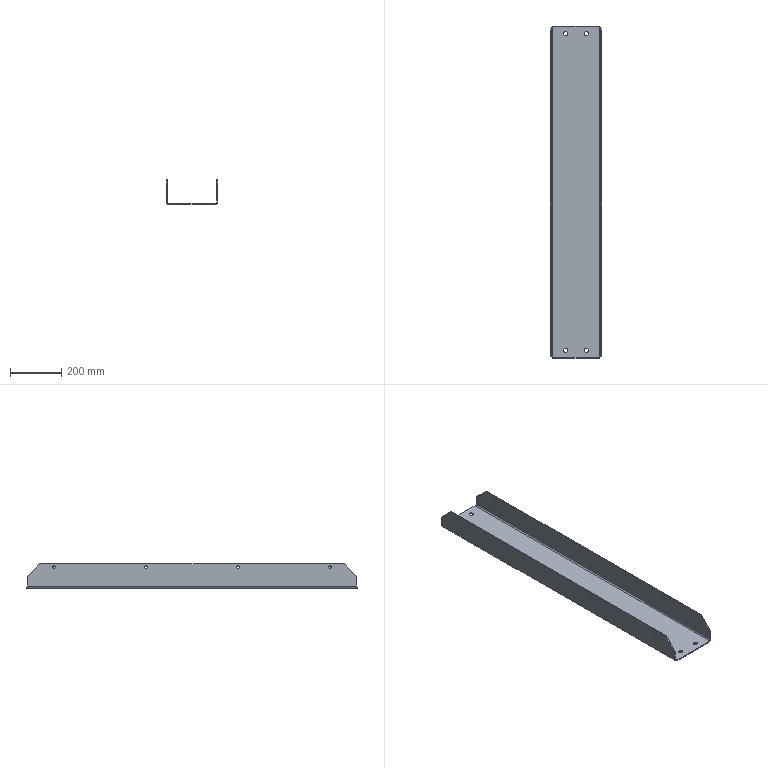Component | SolidWorks | HangingChannelAssembly-2_HangingChannel-1 | 1 solid | 70 faces | volume 1941293 mm3 | cylinder 44 | plane 26 | commonest cylinder face diameters 10 x18 11.5 x8 16 x8 8 x8 18 x2 | material Plain Carbon Steel